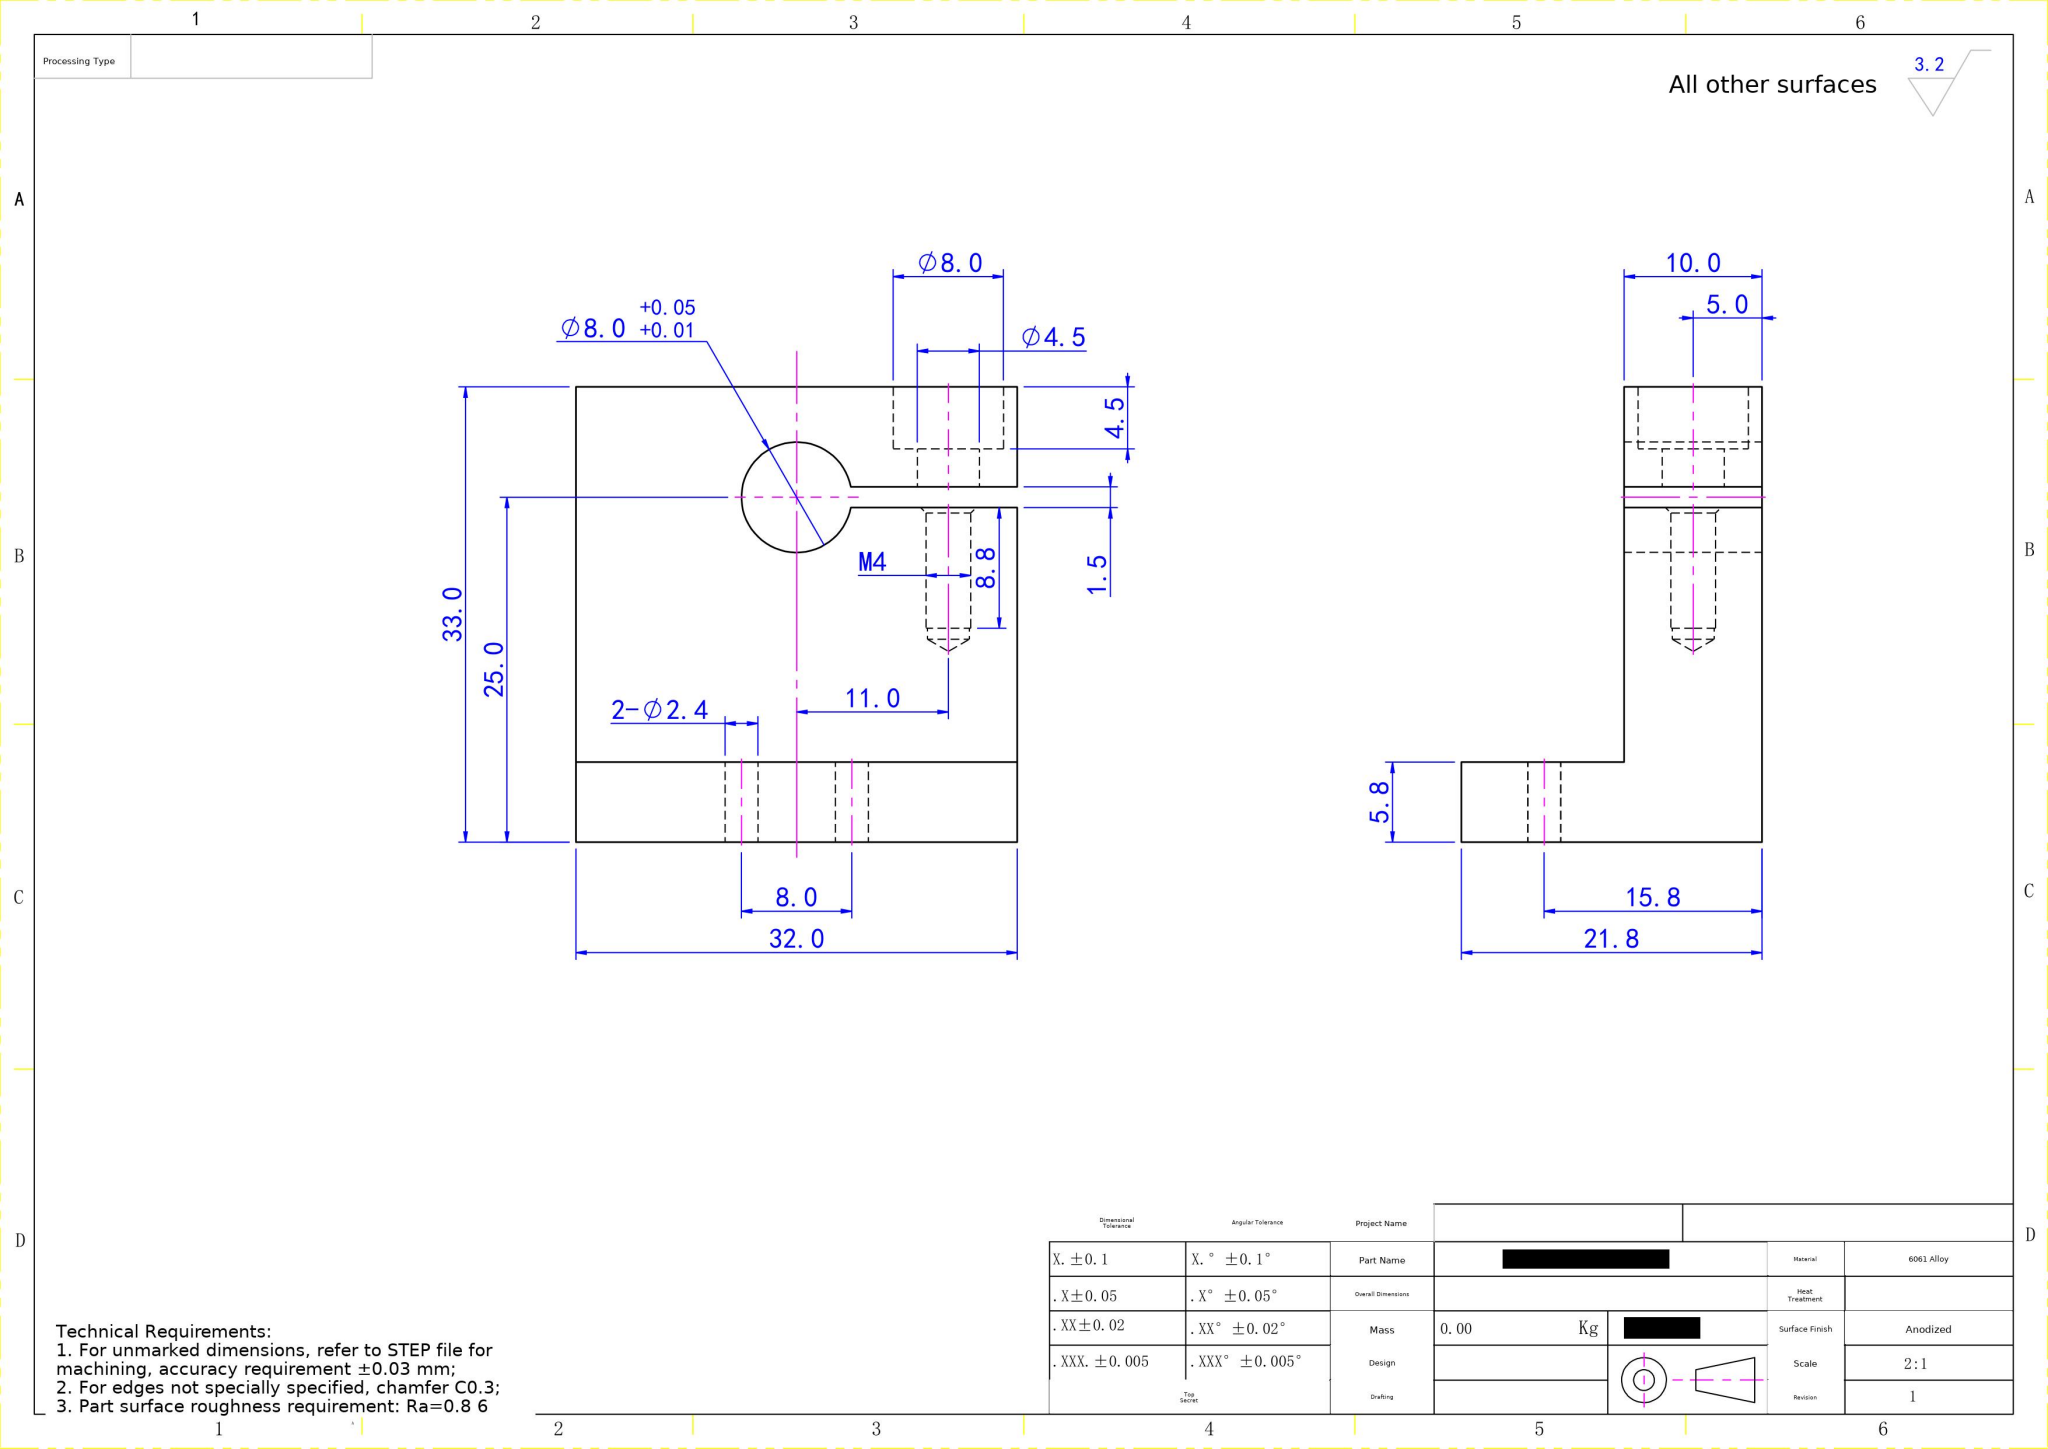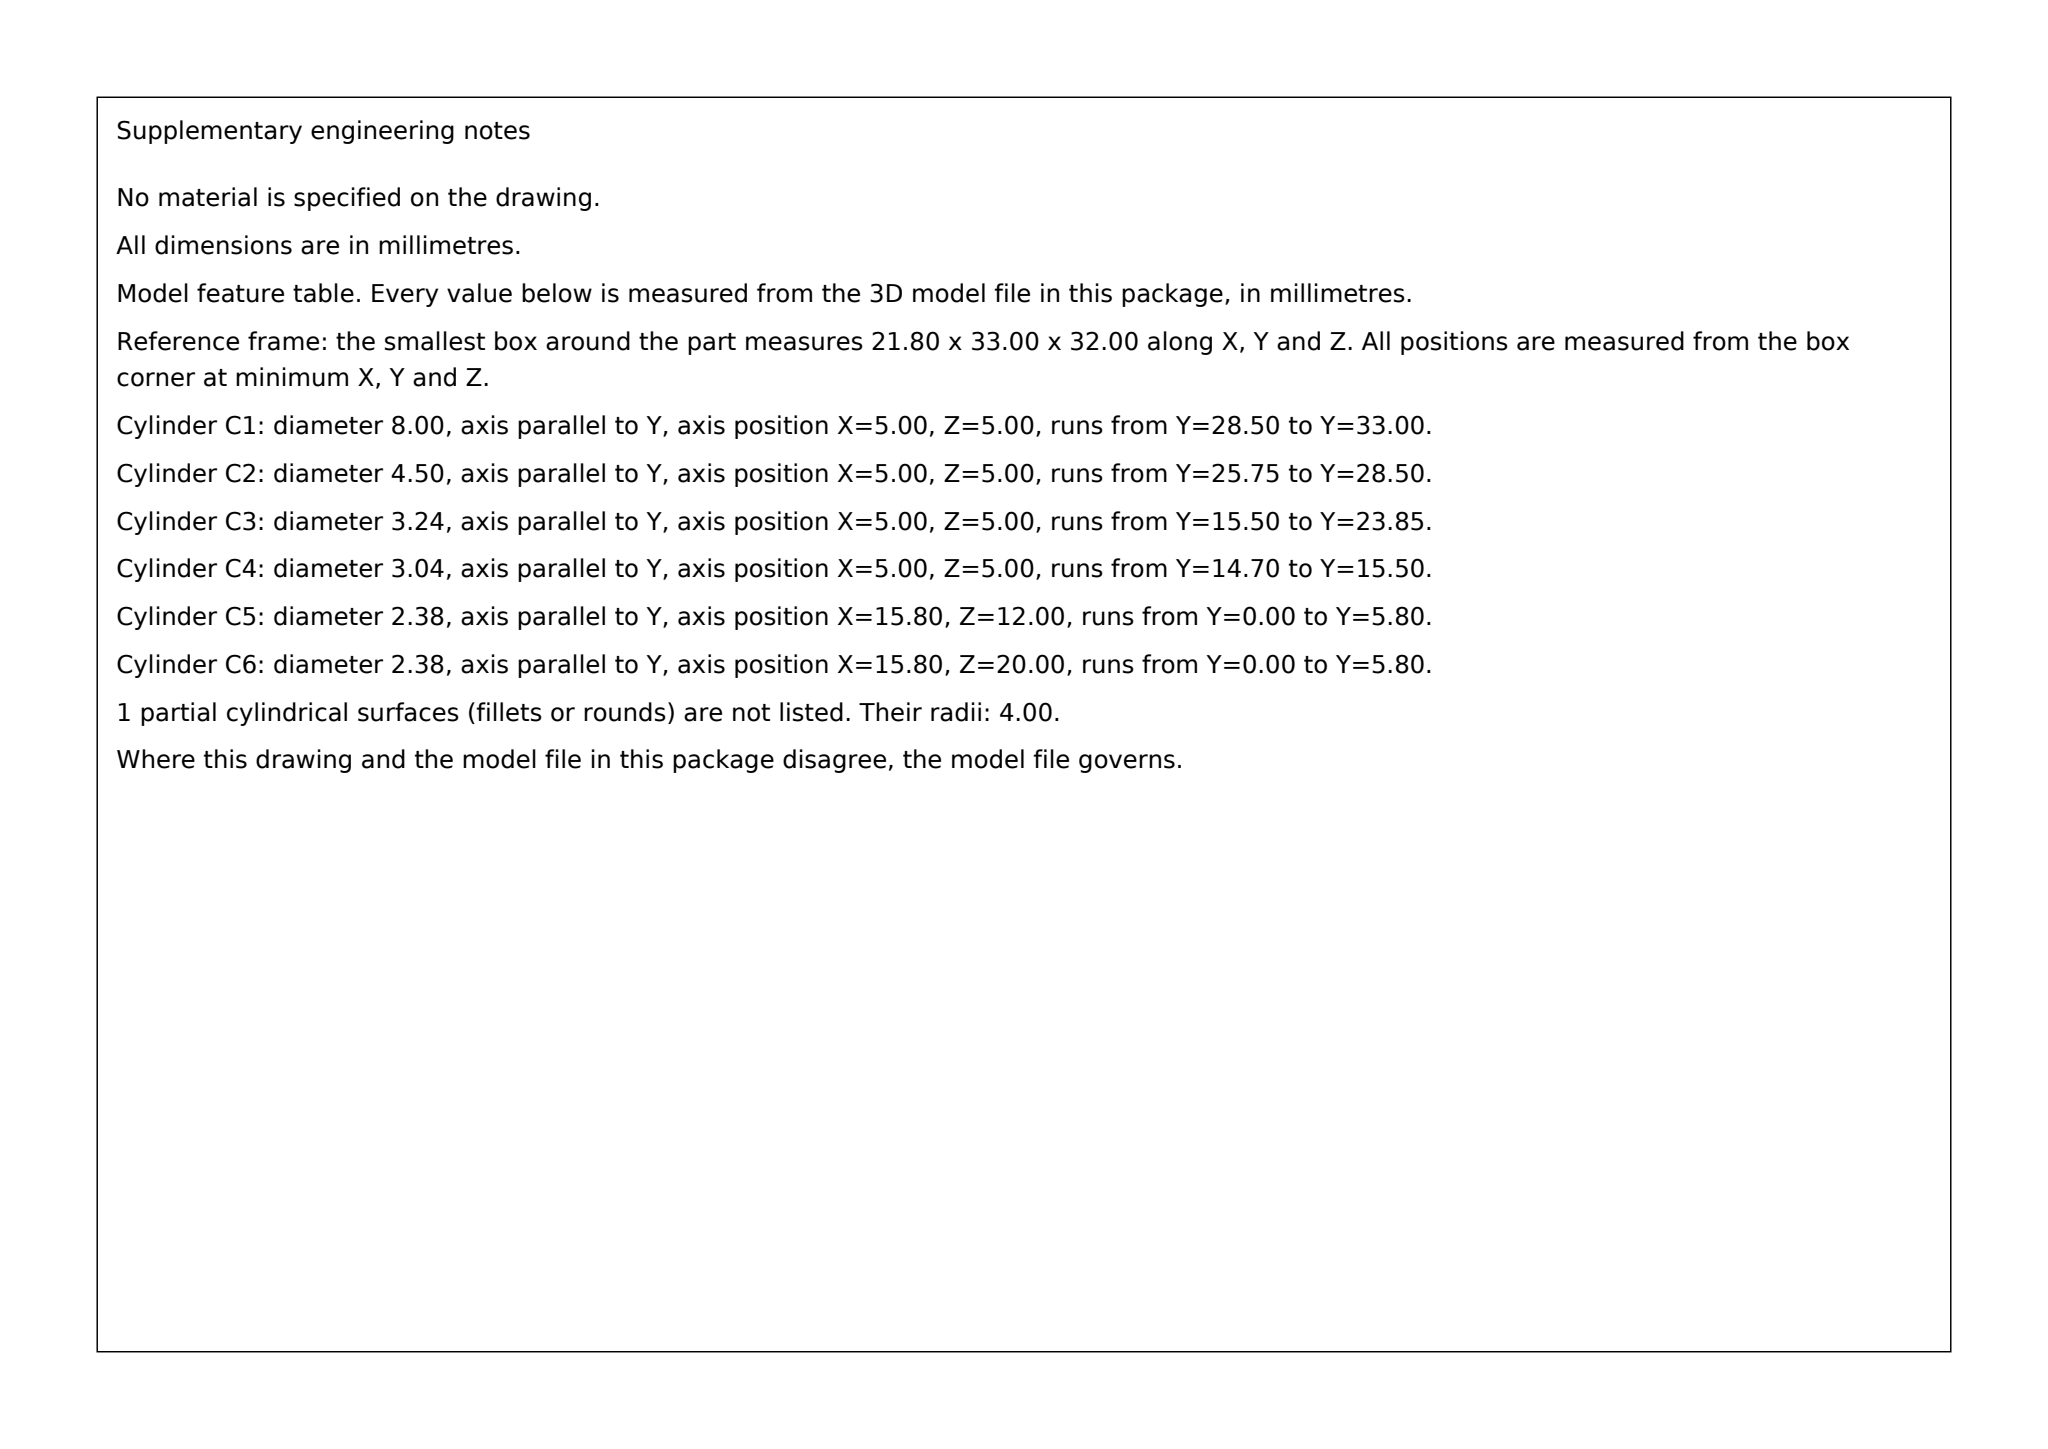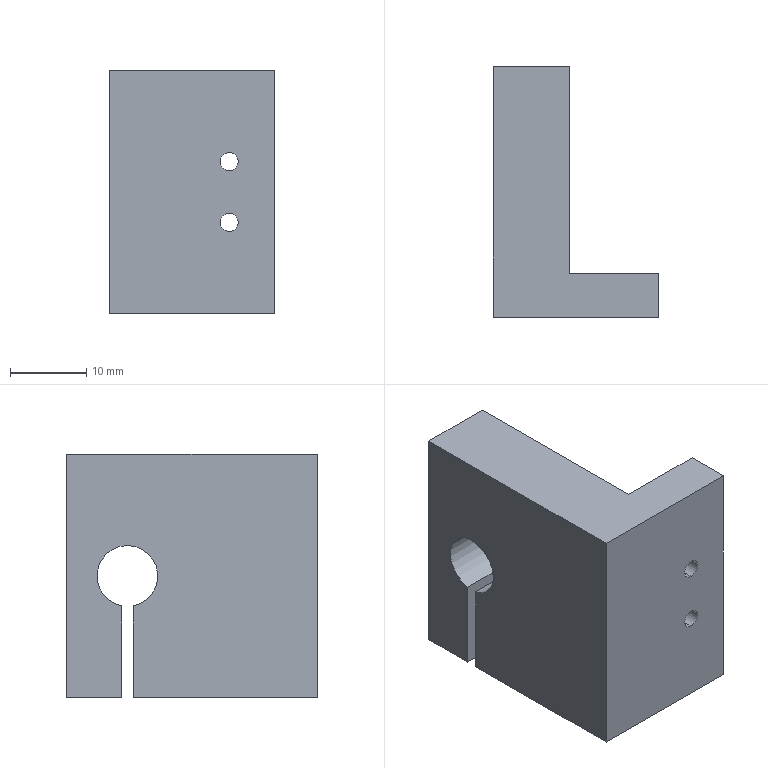Part | SolidWorks | mm | material 6061 Alloy | 1 solid | 31 faces | box 21.8 x 33 x 32 mm | volume 11664 mm3 | cylinder 14 | plane 13 | cone 4 | commonest cylinder face diameters 8 x4 2.389 x2 2.386 x2 3.04 x2 4.5 x2 3.242 x2